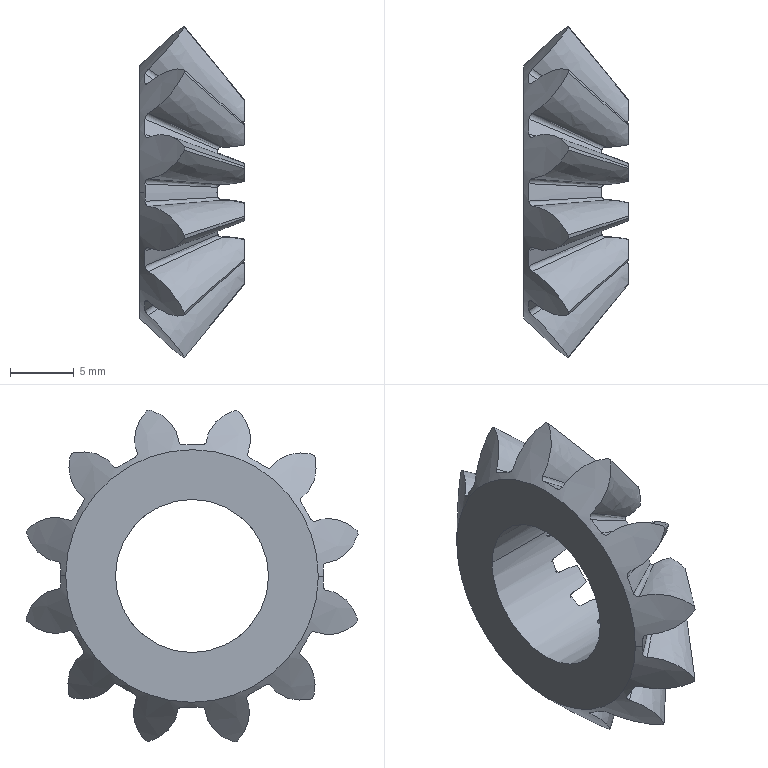Component | SolidWorks | BevelGearNew-12 | 1 solid | 89 faces | volume 1343 mm3 | spline 60 | cone 14 | plane 13 | cylinder 2 | commonest cylinder face diameters 12 x2